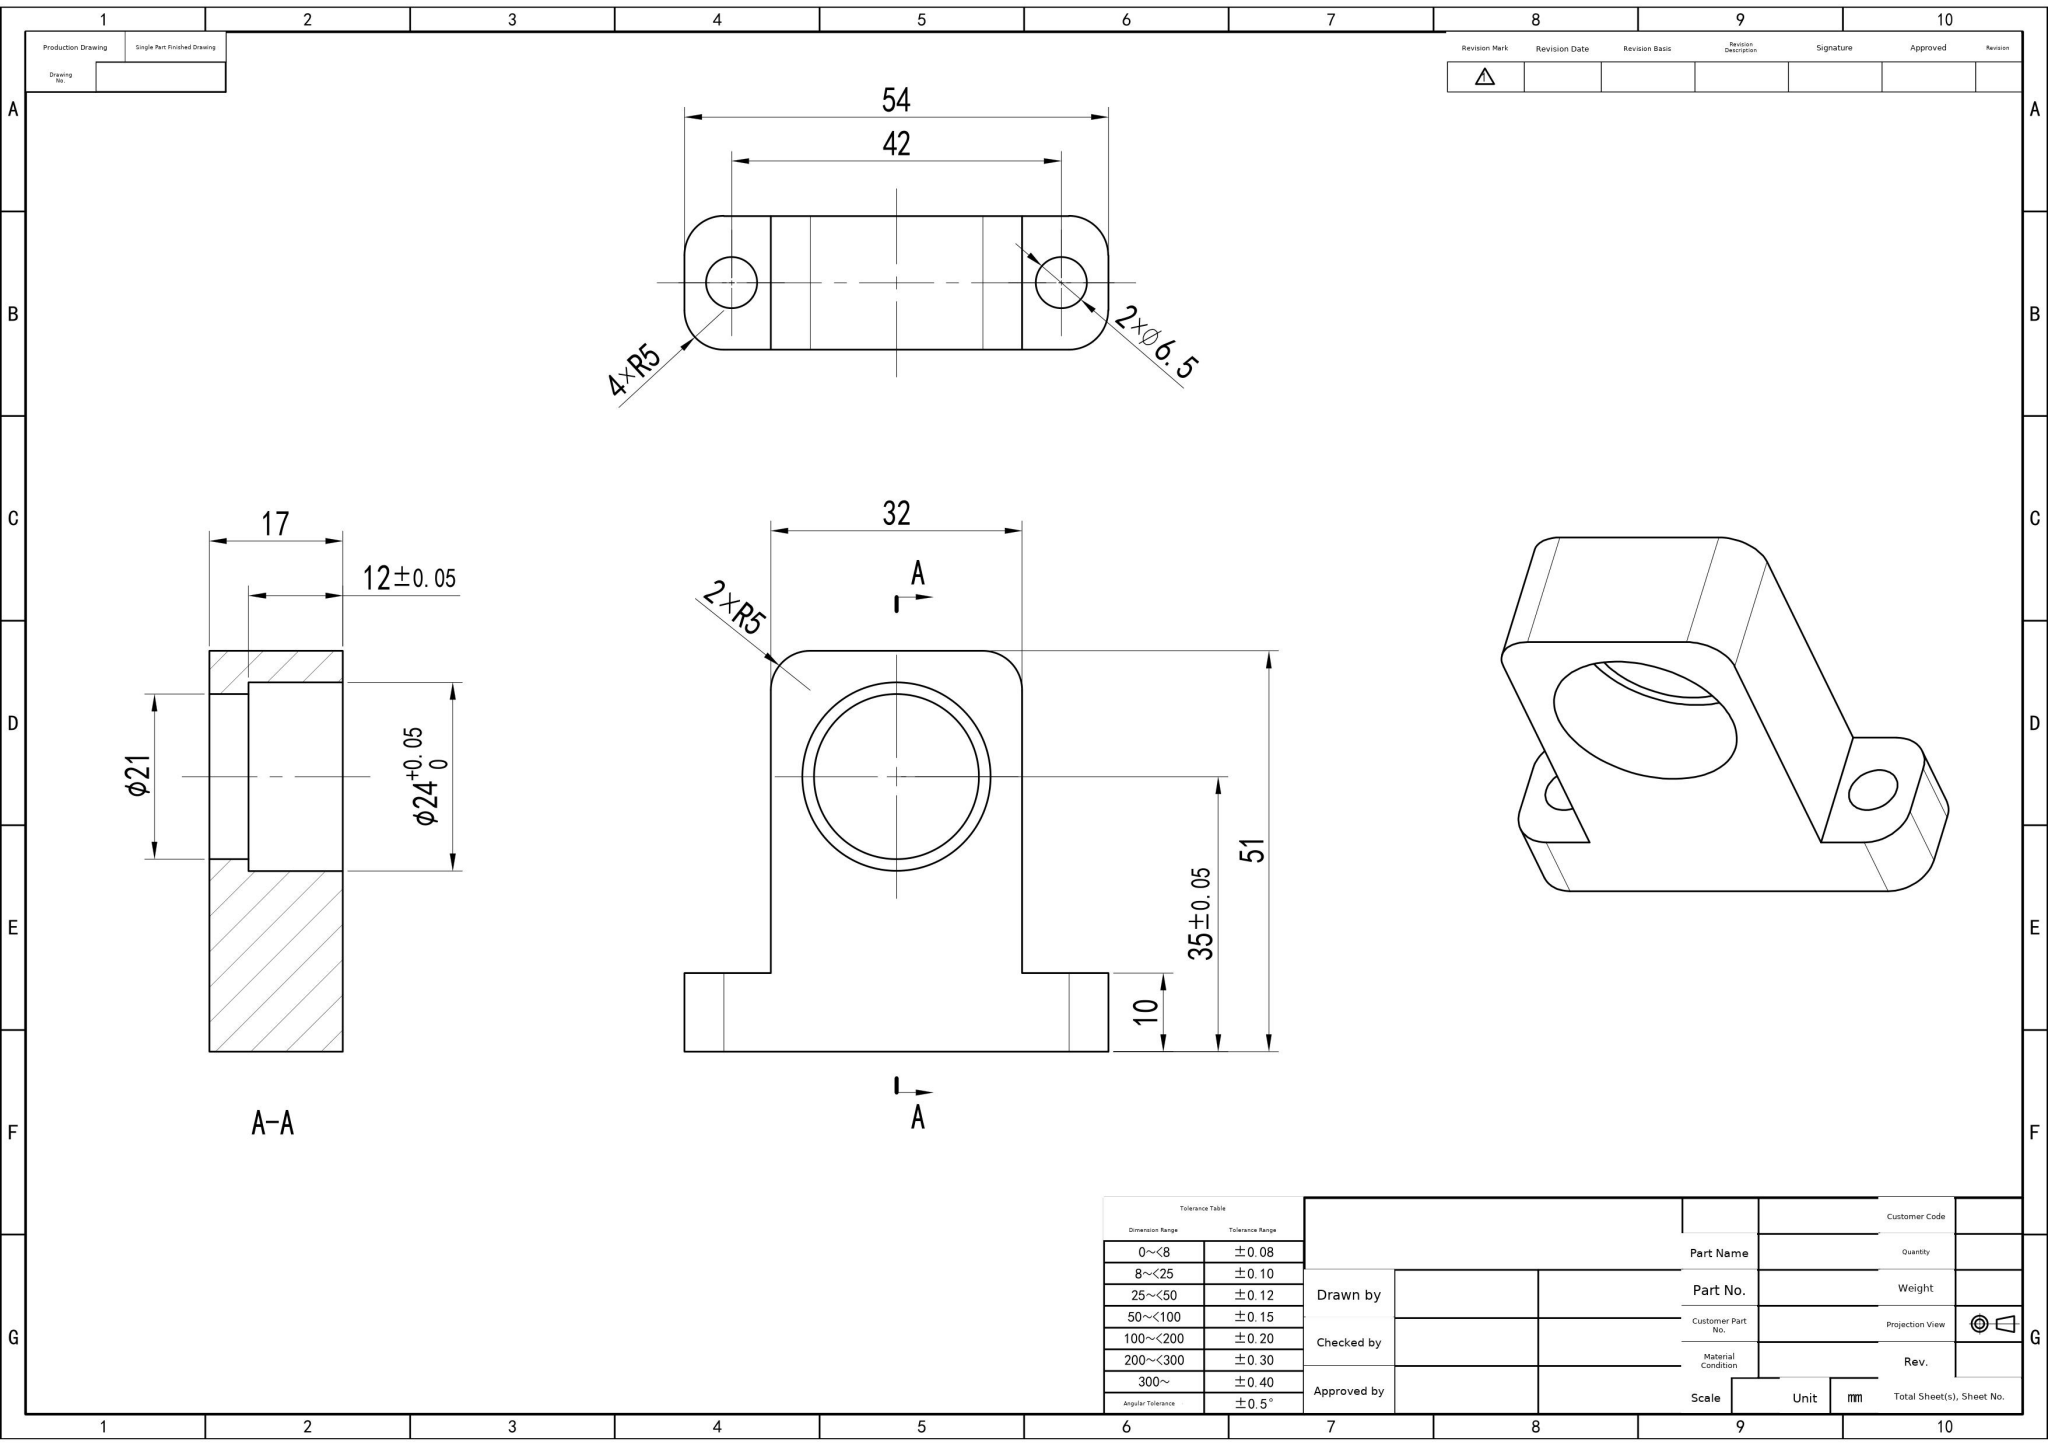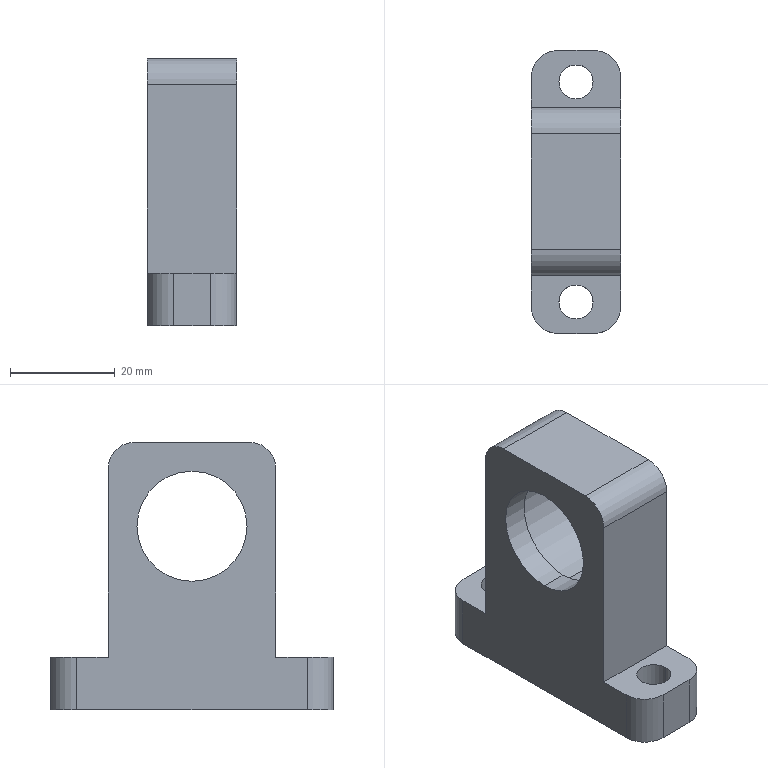Part | SolidWorks | mm | 1 solid | 25 faces | box 17 x 54 x 51 mm | volume 23263 mm3 | cylinder 14 | plane 11 | commonest cylinder face diameters 10 x6 6.5 x4 21 x2 24 x2
STEP:
#1=CARTESIAN_POINT('',(-3.5,0.,24.5));
#2=VERTEX_POINT('',#1);
#3=CARTESIAN_POINT('',(-3.5,0.,45.5));
#4=VERTEX_POINT('',#3);
#5=CARTESIAN_POINT('',(-3.5,0.,35.));
#6=DIRECTION('',(-1.,0.,0.));
#7=DIRECTION('',(0.,0.,1.));
#8=AXIS2_PLACEMENT_3D('',#5,#6,#7);
#9=CIRCLE('',#8,10.5);
#10=EDGE_CURVE('',#2,#4,#9,.T.);
#11=ORIENTED_EDGE('',*,*,#10,.F.);
#12=CARTESIAN_POINT('',(-8.5,0.,24.5));
#13=VERTEX_POINT('',#12);
#14=CARTESIAN_POINT('',(8.5,0.,24.5));
#15=DIRECTION('',(-1.,0.,0.));
#16=VECTOR('',#15,1000.);
#17=LINE('',#14,#16);
#18=EDGE_CURVE('',#2,#13,#17,.T.);
#19=ORIENTED_EDGE('',*,*,#18,.T.);
#20=CARTESIAN_POINT('',(-8.5,0.,45.5));
#21=VERTEX_POINT('',#20);
#22=CARTESIAN_POINT('',(-8.5,0.,35.));
#23=DIRECTION('',(-1.,0.,0.));
#24=DIRECTION('',(0.,0.,1.));
#25=AXIS2_PLACEMENT_3D('',#22,#23,#24);
#26=CIRCLE('',#25,10.5);
#27=EDGE_CURVE('',#13,#21,#26,.T.);
#28=ORIENTED_EDGE('',*,*,#27,.T.);
#29=CARTESIAN_POINT('',(8.5,0.,45.5));
#30=DIRECTION('',(-1.,0.,0.));
#31=VECTOR('',#30,1000.);
#32=LINE('',#29,#31);
#33=EDGE_CURVE('',#4,#21,#32,.T.);
#34=ORIENTED_EDGE('',*,*,#33,.F.);
#35=EDGE_LOOP('',(#11,#19,#28,#34));
#36=FACE_OUTER_BOUND('',#35,.T.);
#37=CARTESIAN_POINT('',(8.5,0.,35.));
#38=DIRECTION('',(-1.,0.,0.));
#39=DIRECTION('',(0.,0.,1.));
#40=AXIS2_PLACEMENT_3D('',#37,#38,#39);
#41=CYLINDRICAL_SURFACE('',#40,10.5);
#42=ADVANCED_FACE('',(#36),#41,.F.);
#43=CARTESIAN_POINT('',(3.25,21.,0.));
#44=VERTEX_POINT('',#43);
#45=CARTESIAN_POINT('',(-3.25,21.,0.));
#46=VERTEX_POINT('',#45);
#47=CARTESIAN_POINT('',(0.,21.,0.));
#48=DIRECTION('',(0.,0.,-1.));
#49=DIRECTION('',(1.,0.,0.));
#50=AXIS2_PLACEMENT_3D('',#47,#48,#49);
#51=CIRCLE('',#50,3.25);
#52=EDGE_CURVE('',#44,#46,#51,.T.);
#53=ORIENTED_EDGE('',*,*,#52,.T.);
#54=CARTESIAN_POINT('',(-3.25,21.,10.));
#55=VERTEX_POINT('',#54);
#56=CARTESIAN_POINT('',(-3.25,21.,0.));
#57=DIRECTION('',(0.,0.,1.));
#58=VECTOR('',#57,1000.);
#59=LINE('',#56,#58);
#60=EDGE_CURVE('',#46,#55,#59,.T.);
#61=ORIENTED_EDGE('',*,*,#60,.T.);
#62=CARTESIAN_POINT('',(3.25,21.,10.));
#63=VERTEX_POINT('',#62);
#64=CARTESIAN_POINT('',(0.,21.,10.));
#65=DIRECTION('',(0.,0.,1.));
#66=DIRECTION('',(1.,0.,0.));
#67=AXIS2_PLACEMENT_3D('',#64,#65,#66);
#68=CIRCLE('',#67,3.25);
#69=EDGE_CURVE('',#55,#63,#68,.T.);
#70=ORIENTED_EDGE('',*,*,#69,.T.);
#71=CARTESIAN_POINT('',(3.25,21.,0.));
#72=DIRECTION('',(0.,0.,1.));
#73=VECTOR('',#72,1000.);
#74=LINE('',#71,#73);
#75=EDGE_CURVE('',#44,#63,#74,.T.);
#76=ORIENTED_EDGE('',*,*,#75,.F.);
#77=EDGE_LOOP('',(#53,#61,#70,#76));
#78=FACE_OUTER_BOUND('',#77,.T.);
#79=CARTESIAN_POINT('',(0.,21.,0.));
#80=DIRECTION('',(0.,0.,1.));
#81=DIRECTION('',(1.,0.,0.));
#82=AXIS2_PLACEMENT_3D('',#79,#80,#81);
#83=CYLINDRICAL_SURFACE('',#82,3.25);
#84=ADVANCED_FACE('',(#78),#83,.F.);
#85=CARTESIAN_POINT('',(3.25,-21.,0.));
#86=VERTEX_POINT('',#85);
#87=CARTESIAN_POINT('',(-3.25,-21.,0.));
#88=VERTEX_POINT('',#87);
#89=CARTESIAN_POINT('',(-0.,-21.,0.));
#90=DIRECTION('',(0.,0.,-1.));
#91=DIRECTION('',(1.,0.,0.));
#92=AXIS2_PLACEMENT_3D('',#89,#90,#91);
#93=CIRCLE('',#92,3.25);
#94=EDGE_CURVE('',#86,#88,#93,.T.);
#95=ORIENTED_EDGE('',*,*,#94,.T.);
#96=CARTESIAN_POINT('',(-3.25,-21.,10.));
#97=VERTEX_POINT('',#96);
#98=CARTESIAN_POINT('',(-3.25,-21.,0.));
#99=DIRECTION('',(0.,0.,1.));
#100=VECTOR('',#99,1000.);
#101=LINE('',#98,#100);
#102=EDGE_CURVE('',#88,#97,#101,.T.);
#103=ORIENTED_EDGE('',*,*,#102,.T.);
#104=CARTESIAN_POINT('',(3.25,-21.,10.));
#105=VERTEX_POINT('',#104);
#106=CARTESIAN_POINT('',(-0.,-21.,10.));
#107=DIRECTION('',(0.,0.,1.));
#108=DIRECTION('',(1.,0.,0.));
#109=AXIS2_PLACEMENT_3D('',#106,#107,#108);
#110=CIRCLE('',#109,3.25);
#111=EDGE_CURVE('',#97,#105,#110,.T.);
#112=ORIENTED_EDGE('',*,*,#111,.T.);
#113=CARTESIAN_POINT('',(3.25,-21.,0.));
#114=DIRECTION('',(0.,0.,1.));
#115=VECTOR('',#114,1000.);
#116=LINE('',#113,#115);
#117=EDGE_CURVE('',#86,#105,#116,.T.);
#118=ORIENTED_EDGE('',*,*,#117,.F.);
#119=EDGE_LOOP('',(#95,#103,#112,#118));
#120=FACE_OUTER_BOUND('',#119,.T.);
#121=CARTESIAN_POINT('',(-0.,-21.,0.));
#122=DIRECTION('',(0.,0.,1.));
#123=DIRECTION('',(1.,0.,0.));
#124=AXIS2_PLACEMENT_3D('',#121,#122,#123);
#125=CYLINDRICAL_SURFACE('',#124,3.25);
#126=ADVANCED_FACE('',(#120),#125,.F.);
#127=CARTESIAN_POINT('',(8.5,0.,23.));
#128=VERTEX_POINT('',#127);
#129=CARTESIAN_POINT('',(8.5,0.,47.));
#130=VERTEX_POINT('',#129);
#131=CARTESIAN_POINT('',(8.5,0.,35.));
#132=DIRECTION('',(-1.,0.,0.));
#133=DIRECTION('',(0.,0.,1.));
#134=AXIS2_PLACEMENT_3D('',#131,#132,#133);
#135=CIRCLE('',#134,12.);
#136=EDGE_CURVE('',#128,#130,#135,.T.);
#137=ORIENTED_EDGE('',*,*,#136,.F.);
#138=CARTESIAN_POINT('',(-3.5,0.,23.));
#139=VERTEX_POINT('',#138);
#140=CARTESIAN_POINT('',(8.5,0.,23.));
#141=DIRECTION('',(-1.,0.,0.));
#142=VECTOR('',#141,1000.);
#143=LINE('',#140,#142);
#144=EDGE_CURVE('',#128,#139,#143,.T.);
#145=ORIENTED_EDGE('',*,*,#144,.T.);
#146=CARTESIAN_POINT('',(-3.5,0.,47.));
#147=VERTEX_POINT('',#146);
#148=CARTESIAN_POINT('',(-3.5,0.,35.));
#149=DIRECTION('',(-1.,0.,0.));
#150=DIRECTION('',(0.,0.,1.));
#151=AXIS2_PLACEMENT_3D('',#148,#149,#150);
#152=CIRCLE('',#151,12.);
#153=EDGE_CURVE('',#139,#147,#152,.T.);
#154=ORIENTED_EDGE('',*,*,#153,.T.);
#155=CARTESIAN_POINT('',(8.5,0.,47.));
#156=DIRECTION('',(-1.,0.,0.));
#157=VECTOR('',#156,1000.);
#158=LINE('',#155,#157);
#159=EDGE_CURVE('',#130,#147,#158,.T.);
#160=ORIENTED_EDGE('',*,*,#159,.F.);
#161=EDGE_LOOP('',(#137,#145,#154,#160));
#162=FACE_OUTER_BOUND('',#161,.T.);
#163=CARTESIAN_POINT('',(8.5,0.,35.));
#164=DIRECTION('',(-1.,0.,0.));
#165=DIRECTION('',(0.,0.,1.));
#166=AXIS2_PLACEMENT_3D('',#163,#164,#165);
#167=CYLINDRICAL_SURFACE('',#166,12.);
#168=ADVANCED_FACE('',(#162),#167,.F.);
#169=CARTESIAN_POINT('',(-8.5,0.,35.));
#170=DIRECTION('',(-1.,0.,0.));
#171=DIRECTION('',(0.,0.,1.));
#172=AXIS2_PLACEMENT_3D('',#169,#170,#171);
#173=CIRCLE('',#172,10.5);
#174=EDGE_CURVE('',#21,#13,#173,.T.);
#175=ORIENTED_EDGE('',*,*,#174,.F.);
#176=ORIENTED_EDGE('',*,*,#27,.F.);
#177=EDGE_LOOP('',(#175,#176));
#178=FACE_BOUND('',#177,.T.);
#179=CARTESIAN_POINT('',(-8.5,22.,-0.));
#180=VERTEX_POINT('',#179);
#181=CARTESIAN_POINT('',(-8.5,22.,10.));
#182=VERTEX_POINT('',#181);
#183=CARTESIAN_POINT('',(-8.5,22.,46.));
#184=DIRECTION('',(0.,0.,1.));
#185=VECTOR('',#184,1000.);
#186=LINE('',#183,#185);
#187=EDGE_CURVE('',#180,#182,#186,.T.);
#188=ORIENTED_EDGE('',*,*,#187,.F.);
#189=CARTESIAN_POINT('',(-8.5,-22.,0.));
#190=VERTEX_POINT('',#189);
#191=CARTESIAN_POINT('',(-8.5,11.,0.));
#192=DIRECTION('',(0.,1.,0.));
#193=VECTOR('',#192,1000.);
#194=LINE('',#191,#193);
#195=EDGE_CURVE('',#190,#180,#194,.T.);
#196=ORIENTED_EDGE('',*,*,#195,.F.);
#197=CARTESIAN_POINT('',(-8.5,-22.,10.));
#198=VERTEX_POINT('',#197);
#199=CARTESIAN_POINT('',(-8.5,-22.,46.));
#200=DIRECTION('',(0.,0.,-1.));
#201=VECTOR('',#200,1000.);
#202=LINE('',#199,#201);
#203=EDGE_CURVE('',#198,#190,#202,.T.);
#204=ORIENTED_EDGE('',*,*,#203,.F.);
#205=CARTESIAN_POINT('',(-8.5,-16.,10.));
#206=VERTEX_POINT('',#205);
#207=CARTESIAN_POINT('',(-8.5,11.,10.));
#208=DIRECTION('',(0.,-1.,0.));
#209=VECTOR('',#208,1000.);
#210=LINE('',#207,#209);
#211=EDGE_CURVE('',#206,#198,#210,.T.);
#212=ORIENTED_EDGE('',*,*,#211,.F.);
#213=CARTESIAN_POINT('',(-8.5,-16.,46.));
#214=VERTEX_POINT('',#213);
#215=CARTESIAN_POINT('',(-8.5,-16.,46.));
#216=DIRECTION('',(0.,0.,-1.));
#217=VECTOR('',#216,1000.);
#218=LINE('',#215,#217);
#219=EDGE_CURVE('',#214,#206,#218,.T.);
#220=ORIENTED_EDGE('',*,*,#219,.F.);
#221=CARTESIAN_POINT('',(-8.5,-11.,51.));
#222=VERTEX_POINT('',#221);
#223=CARTESIAN_POINT('',(-8.5,-11.,46.));
#224=DIRECTION('',(1.,0.,0.));
#225=DIRECTION('',(0.,0.,1.));
#226=AXIS2_PLACEMENT_3D('',#223,#224,#225);
#227=CIRCLE('',#226,5.);
#228=EDGE_CURVE('',#222,#214,#227,.T.);
#229=ORIENTED_EDGE('',*,*,#228,.F.);
#230=CARTESIAN_POINT('',(-8.5,11.,51.));
#231=VERTEX_POINT('',#230);
#232=CARTESIAN_POINT('',(-8.5,11.,51.));
#233=DIRECTION('',(0.,-1.,0.));
#234=VECTOR('',#233,1000.);
#235=LINE('',#232,#234);
#236=EDGE_CURVE('',#231,#222,#235,.T.);
#237=ORIENTED_EDGE('',*,*,#236,.F.);
#238=CARTESIAN_POINT('',(-8.5,16.,46.));
#239=VERTEX_POINT('',#238);
#240=CARTESIAN_POINT('',(-8.5,11.,46.));
#241=DIRECTION('',(1.,0.,0.));
#242=DIRECTION('',(0.,0.,1.));
#243=AXIS2_PLACEMENT_3D('',#240,#241,#242);
#244=CIRCLE('',#243,5.);
#245=EDGE_CURVE('',#239,#231,#244,.T.);
#246=ORIENTED_EDGE('',*,*,#245,.F.);
#247=CARTESIAN_POINT('',(-8.5,16.,10.));
#248=VERTEX_POINT('',#247);
#249=CARTESIAN_POINT('',(-8.5,16.,46.));
#250=DIRECTION('',(0.,0.,1.));
#251=VECTOR('',#250,1000.);
#252=LINE('',#249,#251);
#253=EDGE_CURVE('',#248,#239,#252,.T.);
#254=ORIENTED_EDGE('',*,*,#253,.F.);
#255=CARTESIAN_POINT('',(-8.5,11.,10.));
#256=DIRECTION('',(0.,-1.,0.));
#257=VECTOR('',#256,1000.);
#258=LINE('',#255,#257);
#259=EDGE_CURVE('',#182,#248,#258,.T.);
#260=ORIENTED_EDGE('',*,*,#259,.F.);
#261=EDGE_LOOP('',(#188,#196,#204,#212,#220,#229,#237,#246,#254,#260));
#262=FACE_OUTER_BOUND('',#261,.T.);
#263=CARTESIAN_POINT('',(-8.5,11.,46.));
#264=DIRECTION('',(1.,0.,0.));
#265=DIRECTION('',(0.,0.,-1.));
#266=AXIS2_PLACEMENT_3D('',#263,#264,#265);
#267=PLANE('',#266);
#268=ADVANCED_FACE('',(#178,#262),#267,.F.);
#269=ORIENTED_EDGE('',*,*,#18,.F.);
#270=CARTESIAN_POINT('',(-3.5,0.,35.));
#271=DIRECTION('',(-1.,0.,0.));
#272=DIRECTION('',(0.,0.,1.));
#273=AXIS2_PLACEMENT_3D('',#270,#271,#272);
#274=CIRCLE('',#273,10.5);
#275=EDGE_CURVE('',#4,#2,#274,.T.);
#276=ORIENTED_EDGE('',*,*,#275,.F.);
#277=ORIENTED_EDGE('',*,*,#33,.T.);
#278=ORIENTED_EDGE('',*,*,#174,.T.);
#279=EDGE_LOOP('',(#269,#276,#277,#278));
#280=FACE_OUTER_BOUND('',#279,.T.);
#281=CARTESIAN_POINT('',(8.5,0.,35.));
#282=DIRECTION('',(-1.,0.,0.));
#283=DIRECTION('',(0.,0.,1.));
#284=AXIS2_PLACEMENT_3D('',#281,#282,#283);
#285=CYLINDRICAL_SURFACE('',#284,10.5);
#286=ADVANCED_FACE('',(#280),#285,.F.);
#287=CARTESIAN_POINT('',(3.5,27.,10.));
#288=VERTEX_POINT('',#287);
#289=CARTESIAN_POINT('',(8.5,22.,10.));
#290=VERTEX_POINT('',#289);
#291=CARTESIAN_POINT('',(3.5,22.,10.));
#292=DIRECTION('',(0.,0.,-1.));
#293=DIRECTION('',(0.,1.,0.));
#294=AXIS2_PLACEMENT_3D('',#291,#292,#293);
#295=CIRCLE('',#294,5.);
#296=EDGE_CURVE('',#288,#290,#295,.T.);
#297=ORIENTED_EDGE('',*,*,#296,.F.);
#298=CARTESIAN_POINT('',(-3.5,27.,10.));
#299=VERTEX_POINT('',#298);
#300=CARTESIAN_POINT('',(8.5,27.,10.));
#301=DIRECTION('',(1.,0.,0.));
#302=VECTOR('',#301,1000.);
#303=LINE('',#300,#302);
#304=EDGE_CURVE('',#299,#288,#303,.T.);
#305=ORIENTED_EDGE('',*,*,#304,.F.);
#306=CARTESIAN_POINT('',(-3.5,22.,10.));
#307=DIRECTION('',(0.,0.,-1.));
#308=DIRECTION('',(0.,-1.,-0.));
#309=AXIS2_PLACEMENT_3D('',#306,#307,#308);
#310=CIRCLE('',#309,5.);
#311=EDGE_CURVE('',#182,#299,#310,.T.);
#312=ORIENTED_EDGE('',*,*,#311,.F.);
#313=ORIENTED_EDGE('',*,*,#259,.T.);
#314=CARTESIAN_POINT('',(8.5,16.,10.));
#315=VERTEX_POINT('',#314);
#316=CARTESIAN_POINT('',(8.5,16.,10.));
#317=DIRECTION('',(-1.,0.,0.));
#318=VECTOR('',#317,1000.);
#319=LINE('',#316,#318);
#320=EDGE_CURVE('',#315,#248,#319,.T.);
#321=ORIENTED_EDGE('',*,*,#320,.F.);
#322=CARTESIAN_POINT('',(8.5,27.,10.));
#323=DIRECTION('',(0.,-1.,0.));
#324=VECTOR('',#323,1000.);
#325=LINE('',#322,#324);
#326=EDGE_CURVE('',#290,#315,#325,.T.);
#327=ORIENTED_EDGE('',*,*,#326,.F.);
#328=EDGE_LOOP('',(#297,#305,#312,#313,#321,#327));
#329=FACE_OUTER_BOUND('',#328,.T.);
#330=CARTESIAN_POINT('',(0.,21.,10.));
#331=DIRECTION('',(0.,0.,1.));
#332=DIRECTION('',(1.,0.,0.));
#333=AXIS2_PLACEMENT_3D('',#330,#331,#332);
#334=CIRCLE('',#333,3.25);
#335=EDGE_CURVE('',#63,#55,#334,.T.);
#336=ORIENTED_EDGE('',*,*,#335,.F.);
#337=ORIENTED_EDGE('',*,*,#69,.F.);
#338=EDGE_LOOP('',(#336,#337));
#339=FACE_BOUND('',#338,.T.);
#340=CARTESIAN_POINT('',(8.5,27.,10.));
#341=DIRECTION('',(0.,0.,-1.));
#342=DIRECTION('',(-1.,0.,0.));
#343=AXIS2_PLACEMENT_3D('',#340,#341,#342);
#344=PLANE('',#343);
#345=ADVANCED_FACE('',(#329,#339),#344,.F.);
#346=ORIENTED_EDGE('',*,*,#311,.T.);
#347=CARTESIAN_POINT('',(-3.5,27.,-0.));
#348=VERTEX_POINT('',#347);
#349=CARTESIAN_POINT('',(-3.5,27.,0.));
#350=DIRECTION('',(0.,0.,-1.));
#351=VECTOR('',#350,1000.);
#352=LINE('',#349,#351);
#353=EDGE_CURVE('',#299,#348,#352,.T.);
#354=ORIENTED_EDGE('',*,*,#353,.T.);
#355=CARTESIAN_POINT('',(-3.5,22.,-0.));
#356=DIRECTION('',(0.,-0.,1.));
#357=DIRECTION('',(0.,-1.,-0.));
#358=AXIS2_PLACEMENT_3D('',#355,#356,#357);
#359=CIRCLE('',#358,5.);
#360=EDGE_CURVE('',#348,#180,#359,.T.);
#361=ORIENTED_EDGE('',*,*,#360,.T.);
#362=ORIENTED_EDGE('',*,*,#187,.T.);
#363=EDGE_LOOP('',(#346,#354,#361,#362));
#364=FACE_OUTER_BOUND('',#363,.T.);
#365=CARTESIAN_POINT('',(-3.5,22.,-0.));
#366=DIRECTION('',(0.,-0.,1.));
#367=DIRECTION('',(0.,-1.,-0.));
#368=AXIS2_PLACEMENT_3D('',#365,#366,#367);
#369=CYLINDRICAL_SURFACE('',#368,5.);
#370=ADVANCED_FACE('',(#364),#369,.T.);
#371=CARTESIAN_POINT('',(8.5,22.,0.));
#372=VERTEX_POINT('',#371);
#373=CARTESIAN_POINT('',(3.5,27.,0.));
#374=VERTEX_POINT('',#373);
#375=CARTESIAN_POINT('',(3.5,22.,0.));
#376=DIRECTION('',(0.,-0.,1.));
#377=DIRECTION('',(0.,1.,0.));
#378=AXIS2_PLACEMENT_3D('',#375,#376,#377);
#379=CIRCLE('',#378,5.);
#380=EDGE_CURVE('',#372,#374,#379,.T.);
#381=ORIENTED_EDGE('',*,*,#380,.F.);
#382=CARTESIAN_POINT('',(8.5,-22.,-0.));
#383=VERTEX_POINT('',#382);
#384=CARTESIAN_POINT('',(8.5,-27.,0.));
#385=DIRECTION('',(0.,1.,0.));
#386=VECTOR('',#385,1000.);
#387=LINE('',#384,#386);
#388=EDGE_CURVE('',#383,#372,#387,.T.);
#389=ORIENTED_EDGE('',*,*,#388,.F.);
#390=CARTESIAN_POINT('',(3.5,-27.,-0.));
#391=VERTEX_POINT('',#390);
#392=CARTESIAN_POINT('',(3.5,-22.,-0.));
#393=DIRECTION('',(0.,0.,1.));
#394=DIRECTION('',(0.,-1.,0.));
#395=AXIS2_PLACEMENT_3D('',#392,#393,#394);
#396=CIRCLE('',#395,5.);
#397=EDGE_CURVE('',#391,#383,#396,.T.);
#398=ORIENTED_EDGE('',*,*,#397,.F.);
#399=CARTESIAN_POINT('',(-3.5,-27.,0.));
#400=VERTEX_POINT('',#399);
#401=CARTESIAN_POINT('',(8.5,-27.,0.));
#402=DIRECTION('',(1.,0.,0.));
#403=VECTOR('',#402,1000.);
#404=LINE('',#401,#403);
#405=EDGE_CURVE('',#400,#391,#404,.T.);
#406=ORIENTED_EDGE('',*,*,#405,.F.);
#407=CARTESIAN_POINT('',(-3.5,-22.,0.));
#408=DIRECTION('',(0.,0.,1.));
#409=DIRECTION('',(0.,1.,-0.));
#410=AXIS2_PLACEMENT_3D('',#407,#408,#409);
#411=CIRCLE('',#410,5.);
#412=EDGE_CURVE('',#190,#400,#411,.T.);
#413=ORIENTED_EDGE('',*,*,#412,.F.);
#414=ORIENTED_EDGE('',*,*,#195,.T.);
#415=ORIENTED_EDGE('',*,*,#360,.F.);
#416=CARTESIAN_POINT('',(8.5,27.,0.));
#417=DIRECTION('',(-1.,0.,0.));
#418=VECTOR('',#417,1000.);
#419=LINE('',#416,#418);
#420=EDGE_CURVE('',#374,#348,#419,.T.);
#421=ORIENTED_EDGE('',*,*,#420,.F.);
#422=EDGE_LOOP('',(#381,#389,#398,#406,#413,#414,#415,#421));
#423=FACE_OUTER_BOUND('',#422,.T.);
#424=ORIENTED_EDGE('',*,*,#94,.F.);
#425=CARTESIAN_POINT('',(-0.,-21.,0.));
#426=DIRECTION('',(0.,0.,-1.));
#427=DIRECTION('',(1.,0.,0.));
#428=AXIS2_PLACEMENT_3D('',#425,#426,#427);
#429=CIRCLE('',#428,3.25);
#430=EDGE_CURVE('',#88,#86,#429,.T.);
#431=ORIENTED_EDGE('',*,*,#430,.F.);
#432=EDGE_LOOP('',(#424,#431));
#433=FACE_BOUND('',#432,.T.);
#434=ORIENTED_EDGE('',*,*,#52,.F.);
#435=CARTESIAN_POINT('',(0.,21.,0.));
#436=DIRECTION('',(0.,0.,-1.));
#437=DIRECTION('',(1.,0.,0.));
#438=AXIS2_PLACEMENT_3D('',#435,#436,#437);
#439=CIRCLE('',#438,3.25);
#440=EDGE_CURVE('',#46,#44,#439,.T.);
#441=ORIENTED_EDGE('',*,*,#440,.F.);
#442=EDGE_LOOP('',(#434,#441));
#443=FACE_BOUND('',#442,.T.);
#444=CARTESIAN_POINT('',(8.5,-27.,0.));
#445=DIRECTION('',(0.,0.,1.));
#446=DIRECTION('',(1.,0.,0.));
#447=AXIS2_PLACEMENT_3D('',#444,#445,#446);
#448=PLANE('',#447);
#449=ADVANCED_FACE('',(#423,#433,#443),#448,.F.);
#450=ORIENTED_EDGE('',*,*,#412,.T.);
#451=CARTESIAN_POINT('',(-3.5,-27.,10.));
#452=VERTEX_POINT('',#451);
#453=CARTESIAN_POINT('',(-3.5,-27.,10.));
#454=DIRECTION('',(0.,0.,1.));
#455=VECTOR('',#454,1000.);
#456=LINE('',#453,#455);
#457=EDGE_CURVE('',#400,#452,#456,.T.);
#458=ORIENTED_EDGE('',*,*,#457,.T.);
#459=CARTESIAN_POINT('',(-3.5,-22.,10.));
#460=DIRECTION('',(0.,-0.,-1.));
#461=DIRECTION('',(0.,1.,-0.));
#462=AXIS2_PLACEMENT_3D('',#459,#460,#461);
#463=CIRCLE('',#462,5.);
#464=EDGE_CURVE('',#452,#198,#463,.T.);
#465=ORIENTED_EDGE('',*,*,#464,.T.);
#466=ORIENTED_EDGE('',*,*,#203,.T.);
#467=EDGE_LOOP('',(#450,#458,#465,#466));
#468=FACE_OUTER_BOUND('',#467,.T.);
#469=CARTESIAN_POINT('',(-3.5,-22.,10.));
#470=DIRECTION('',(0.,-0.,-1.));
#471=DIRECTION('',(0.,1.,-0.));
#472=AXIS2_PLACEMENT_3D('',#469,#470,#471);
#473=CYLINDRICAL_SURFACE('',#472,5.);
#474=ADVANCED_FACE('',(#468),#473,.T.);
#475=CARTESIAN_POINT('',(8.5,-22.,10.));
#476=VERTEX_POINT('',#475);
#477=CARTESIAN_POINT('',(3.5,-27.,10.));
#478=VERTEX_POINT('',#477);
#479=CARTESIAN_POINT('',(3.5,-22.,10.));
#480=DIRECTION('',(0.,-0.,-1.));
#481=DIRECTION('',(-0.,-1.,0.));
#482=AXIS2_PLACEMENT_3D('',#479,#480,#481);
#483=CIRCLE('',#482,5.);
#484=EDGE_CURVE('',#476,#478,#483,.T.);
#485=ORIENTED_EDGE('',*,*,#484,.F.);
#486=CARTESIAN_POINT('',(8.5,-16.,10.));
#487=VERTEX_POINT('',#486);
#488=CARTESIAN_POINT('',(8.5,-16.,10.));
#489=DIRECTION('',(0.,-1.,0.));
#490=VECTOR('',#489,1000.);
#491=LINE('',#488,#490);
#492=EDGE_CURVE('',#487,#476,#491,.T.);
#493=ORIENTED_EDGE('',*,*,#492,.F.);
#494=CARTESIAN_POINT('',(8.5,-16.,10.));
#495=DIRECTION('',(1.,0.,0.));
#496=VECTOR('',#495,1000.);
#497=LINE('',#494,#496);
#498=EDGE_CURVE('',#206,#487,#497,.T.);
#499=ORIENTED_EDGE('',*,*,#498,.F.);
#500=ORIENTED_EDGE('',*,*,#211,.T.);
#501=ORIENTED_EDGE('',*,*,#464,.F.);
#502=CARTESIAN_POINT('',(8.5,-27.,10.));
#503=DIRECTION('',(-1.,0.,0.));
#504=VECTOR('',#503,1000.);
#505=LINE('',#502,#504);
#506=EDGE_CURVE('',#478,#452,#505,.T.);
#507=ORIENTED_EDGE('',*,*,#506,.F.);
#508=EDGE_LOOP('',(#485,#493,#499,#500,#501,#507));
#509=FACE_OUTER_BOUND('',#508,.T.);
#510=CARTESIAN_POINT('',(-0.,-21.,10.));
#511=DIRECTION('',(0.,0.,1.));
#512=DIRECTION('',(1.,0.,0.));
#513=AXIS2_PLACEMENT_3D('',#510,#511,#512);
#514=CIRCLE('',#513,3.25);
#515=EDGE_CURVE('',#105,#97,#514,.T.);
#516=ORIENTED_EDGE('',*,*,#515,.F.);
#517=ORIENTED_EDGE('',*,*,#111,.F.);
#518=EDGE_LOOP('',(#516,#517));
#519=FACE_BOUND('',#518,.T.);
#520=CARTESIAN_POINT('',(8.5,-16.,10.));
#521=DIRECTION('',(0.,0.,-1.));
#522=DIRECTION('',(-1.,0.,0.));
#523=AXIS2_PLACEMENT_3D('',#520,#521,#522);
#524=PLANE('',#523);
#525=ADVANCED_FACE('',(#509,#519),#524,.F.);
#526=ORIENTED_EDGE('',*,*,#498,.T.);
#527=CARTESIAN_POINT('',(8.5,-16.,46.));
#528=VERTEX_POINT('',#527);
#529=CARTESIAN_POINT('',(8.5,-16.,46.));
#530=DIRECTION('',(0.,0.,-1.));
#531=VECTOR('',#530,1000.);
#532=LINE('',#529,#531);
#533=EDGE_CURVE('',#528,#487,#532,.T.);
#534=ORIENTED_EDGE('',*,*,#533,.F.);
#535=CARTESIAN_POINT('',(8.5,-16.,46.));
#536=DIRECTION('',(1.,0.,0.));
#537=VECTOR('',#536,1000.);
#538=LINE('',#535,#537);
#539=EDGE_CURVE('',#214,#528,#538,.T.);
#540=ORIENTED_EDGE('',*,*,#539,.F.);
#541=ORIENTED_EDGE('',*,*,#219,.T.);
#542=EDGE_LOOP('',(#526,#534,#540,#541));
#543=FACE_OUTER_BOUND('',#542,.T.);
#544=CARTESIAN_POINT('',(8.5,-16.,46.));
#545=DIRECTION('',(0.,1.,0.));
#546=DIRECTION('',(0.,0.,1.));
#547=AXIS2_PLACEMENT_3D('',#544,#545,#546);
#548=PLANE('',#547);
#549=ADVANCED_FACE('',(#543),#548,.F.);
#550=CARTESIAN_POINT('',(8.5,-11.,51.));
#551=VERTEX_POINT('',#550);
#552=CARTESIAN_POINT('',(8.5,-11.,46.));
#553=DIRECTION('',(-1.,0.,0.));
#554=DIRECTION('',(0.,0.,1.));
#555=AXIS2_PLACEMENT_3D('',#552,#553,#554);
#556=CIRCLE('',#555,5.);
#557=EDGE_CURVE('',#528,#551,#556,.T.);
#558=ORIENTED_EDGE('',*,*,#557,.T.);
#559=CARTESIAN_POINT('',(8.5,-11.,51.));
#560=DIRECTION('',(-1.,0.,0.));
#561=VECTOR('',#560,1000.);
#562=LINE('',#559,#561);
#563=EDGE_CURVE('',#551,#222,#562,.T.);
#564=ORIENTED_EDGE('',*,*,#563,.T.);
#565=ORIENTED_EDGE('',*,*,#228,.T.);
#566=ORIENTED_EDGE('',*,*,#539,.T.);
#567=EDGE_LOOP('',(#558,#564,#565,#566));
#568=FACE_OUTER_BOUND('',#567,.T.);
#569=CARTESIAN_POINT('',(8.5,-11.,46.));
#570=DIRECTION('',(-1.,0.,0.));
#571=DIRECTION('',(0.,0.,1.));
#572=AXIS2_PLACEMENT_3D('',#569,#570,#571);
#573=CYLINDRICAL_SURFACE('',#572,5.);
#574=ADVANCED_FACE('',(#568),#573,.T.);
#575=ORIENTED_EDGE('',*,*,#563,.F.);
#576=CARTESIAN_POINT('',(8.5,11.,51.));
#577=VERTEX_POINT('',#576);
#578=CARTESIAN_POINT('',(8.5,11.,51.));
#579=DIRECTION('',(0.,-1.,0.));
#580=VECTOR('',#579,1000.);
#581=LINE('',#578,#580);
#582=EDGE_CURVE('',#577,#551,#581,.T.);
#583=ORIENTED_EDGE('',*,*,#582,.F.);
#584=CARTESIAN_POINT('',(8.5,11.,51.));
#585=DIRECTION('',(1.,0.,0.));
#586=VECTOR('',#585,1000.);
#587=LINE('',#584,#586);
#588=EDGE_CURVE('',#231,#577,#587,.T.);
#589=ORIENTED_EDGE('',*,*,#588,.F.);
#590=ORIENTED_EDGE('',*,*,#236,.T.);
#591=EDGE_LOOP('',(#575,#583,#589,#590));
#592=FACE_OUTER_BOUND('',#591,.T.);
#593=CARTESIAN_POINT('',(8.5,11.,51.));
#594=DIRECTION('',(0.,-0.,-1.));
#595=DIRECTION('',(0.,1.,-0.));
#596=AXIS2_PLACEMENT_3D('',#593,#594,#595);
#597=PLANE('',#596);
#598=ADVANCED_FACE('',(#592),#597,.F.);
#599=CARTESIAN_POINT('',(8.5,16.,46.));
#600=VERTEX_POINT('',#599);
#601=CARTESIAN_POINT('',(8.5,11.,46.));
#602=DIRECTION('',(-1.,0.,0.));
#603=DIRECTION('',(0.,0.,1.));
#604=AXIS2_PLACEMENT_3D('',#601,#602,#603);
#605=CIRCLE('',#604,5.);
#606=EDGE_CURVE('',#577,#600,#605,.T.);
#607=ORIENTED_EDGE('',*,*,#606,.T.);
#608=CARTESIAN_POINT('',(8.5,16.,46.));
#609=DIRECTION('',(-1.,0.,0.));
#610=VECTOR('',#609,1000.);
#611=LINE('',#608,#610);
#612=EDGE_CURVE('',#600,#239,#611,.T.);
#613=ORIENTED_EDGE('',*,*,#612,.T.);
#614=ORIENTED_EDGE('',*,*,#245,.T.);
#615=ORIENTED_EDGE('',*,*,#588,.T.);
#616=EDGE_LOOP('',(#607,#613,#614,#615));
#617=FACE_OUTER_BOUND('',#616,.T.);
#618=CARTESIAN_POINT('',(8.5,11.,46.));
#619=DIRECTION('',(-1.,0.,0.));
#620=DIRECTION('',(0.,0.,1.));
#621=AXIS2_PLACEMENT_3D('',#618,#619,#620);
#622=CYLINDRICAL_SURFACE('',#621,5.);
#623=ADVANCED_FACE('',(#617),#622,.T.);
#624=ORIENTED_EDGE('',*,*,#612,.F.);
#625=CARTESIAN_POINT('',(8.5,16.,10.));
#626=DIRECTION('',(0.,0.,1.));
#627=VECTOR('',#626,1000.);
#628=LINE('',#625,#627);
#629=EDGE_CURVE('',#315,#600,#628,.T.);
#630=ORIENTED_EDGE('',*,*,#629,.F.);
#631=ORIENTED_EDGE('',*,*,#320,.T.);
#632=ORIENTED_EDGE('',*,*,#253,.T.);
#633=EDGE_LOOP('',(#624,#630,#631,#632));
#634=FACE_OUTER_BOUND('',#633,.T.);
#635=CARTESIAN_POINT('',(8.5,16.,10.));
#636=DIRECTION('',(0.,-1.,0.));
#637=DIRECTION('',(0.,0.,-1.));
#638=AXIS2_PLACEMENT_3D('',#635,#636,#637);
#639=PLANE('',#638);
#640=ADVANCED_FACE('',(#634),#639,.F.);
#641=CARTESIAN_POINT('',(-3.5,0.,35.));
#642=DIRECTION('',(-1.,0.,0.));
#643=DIRECTION('',(0.,0.,1.));
#644=AXIS2_PLACEMENT_3D('',#641,#642,#643);
#645=CIRCLE('',#644,12.);
#646=EDGE_CURVE('',#147,#139,#645,.T.);
#647=ORIENTED_EDGE('',*,*,#646,.F.);
#648=ORIENTED_EDGE('',*,*,#153,.F.);
#649=EDGE_LOOP('',(#647,#648));
#650=FACE_OUTER_BOUND('',#649,.T.);
#651=ORIENTED_EDGE('',*,*,#275,.T.);
#652=ORIENTED_EDGE('',*,*,#10,.T.);
#653=EDGE_LOOP('',(#651,#652));
#654=FACE_BOUND('',#653,.T.);
#655=CARTESIAN_POINT('',(-3.5,0.,35.));
#656=DIRECTION('',(-1.,0.,0.));
#657=DIRECTION('',(0.,0.,1.));
#658=AXIS2_PLACEMENT_3D('',#655,#656,#657);
#659=PLANE('',#658);
#660=ADVANCED_FACE('',(#650,#654),#659,.F.);
#661=ORIENTED_EDGE('',*,*,#492,.T.);
#662=CARTESIAN_POINT('',(8.5,-22.,46.));
#663=DIRECTION('',(0.,0.,-1.));
#664=VECTOR('',#663,1000.);
#665=LINE('',#662,#664);
#666=EDGE_CURVE('',#476,#383,#665,.T.);
#667=ORIENTED_EDGE('',*,*,#666,.T.);
#668=ORIENTED_EDGE('',*,*,#388,.T.);
#669=CARTESIAN_POINT('',(8.5,22.,46.));
#670=DIRECTION('',(0.,0.,1.));
#671=VECTOR('',#670,1000.);
#672=LINE('',#669,#671);
#673=EDGE_CURVE('',#372,#290,#672,.T.);
#674=ORIENTED_EDGE('',*,*,#673,.T.);
#675=ORIENTED_EDGE('',*,*,#326,.T.);
#676=ORIENTED_EDGE('',*,*,#629,.T.);
#677=ORIENTED_EDGE('',*,*,#606,.F.);
#678=ORIENTED_EDGE('',*,*,#582,.T.);
#679=ORIENTED_EDGE('',*,*,#557,.F.);
#680=ORIENTED_EDGE('',*,*,#533,.T.);
#681=EDGE_LOOP('',(#661,#667,#668,#674,#675,#676,#677,#678,#679,#680));
#682=FACE_OUTER_BOUND('',#681,.T.);
#683=CARTESIAN_POINT('',(8.5,0.,35.));
#684=DIRECTION('',(-1.,0.,0.));
#685=DIRECTION('',(0.,0.,1.));
#686=AXIS2_PLACEMENT_3D('',#683,#684,#685);
#687=CIRCLE('',#686,12.);
#688=EDGE_CURVE('',#130,#128,#687,.T.);
#689=ORIENTED_EDGE('',*,*,#688,.T.);
#690=ORIENTED_EDGE('',*,*,#136,.T.);
#691=EDGE_LOOP('',(#689,#690));
#692=FACE_BOUND('',#691,.T.);
#693=CARTESIAN_POINT('',(8.5,11.,46.));
#694=DIRECTION('',(1.,0.,0.));
#695=DIRECTION('',(0.,0.,-1.));
#696=AXIS2_PLACEMENT_3D('',#693,#694,#695);
#697=PLANE('',#696);
#698=ADVANCED_FACE('',(#682,#692),#697,.T.);
#699=ORIENTED_EDGE('',*,*,#296,.T.);
#700=ORIENTED_EDGE('',*,*,#673,.F.);
#701=ORIENTED_EDGE('',*,*,#380,.T.);
#702=CARTESIAN_POINT('',(3.5,27.,46.));
#703=DIRECTION('',(0.,-0.,1.));
#704=VECTOR('',#703,1000.);
#705=LINE('',#702,#704);
#706=EDGE_CURVE('',#374,#288,#705,.T.);
#707=ORIENTED_EDGE('',*,*,#706,.T.);
#708=EDGE_LOOP('',(#699,#700,#701,#707));
#709=FACE_OUTER_BOUND('',#708,.T.);
#710=CARTESIAN_POINT('',(3.5,22.,46.));
#711=DIRECTION('',(0.,0.,-1.));
#712=DIRECTION('',(0.,1.,0.));
#713=AXIS2_PLACEMENT_3D('',#710,#711,#712);
#714=CYLINDRICAL_SURFACE('',#713,5.);
#715=ADVANCED_FACE('',(#709),#714,.T.);
#716=ORIENTED_EDGE('',*,*,#706,.F.);
#717=ORIENTED_EDGE('',*,*,#420,.T.);
#718=ORIENTED_EDGE('',*,*,#353,.F.);
#719=ORIENTED_EDGE('',*,*,#304,.T.);
#720=EDGE_LOOP('',(#716,#717,#718,#719));
#721=FACE_OUTER_BOUND('',#720,.T.);
#722=CARTESIAN_POINT('',(8.5,27.,0.));
#723=DIRECTION('',(0.,-1.,-0.));
#724=DIRECTION('',(0.,0.,-1.));
#725=AXIS2_PLACEMENT_3D('',#722,#723,#724);
#726=PLANE('',#725);
#727=ADVANCED_FACE('',(#721),#726,.F.);
#728=ORIENTED_EDGE('',*,*,#60,.F.);
#729=ORIENTED_EDGE('',*,*,#440,.T.);
#730=ORIENTED_EDGE('',*,*,#75,.T.);
#731=ORIENTED_EDGE('',*,*,#335,.T.);
#732=EDGE_LOOP('',(#728,#729,#730,#731));
#733=FACE_OUTER_BOUND('',#732,.T.);
#734=CARTESIAN_POINT('',(0.,21.,0.));
#735=DIRECTION('',(0.,0.,1.));
#736=DIRECTION('',(1.,0.,0.));
#737=AXIS2_PLACEMENT_3D('',#734,#735,#736);
#738=CYLINDRICAL_SURFACE('',#737,3.25);
#739=ADVANCED_FACE('',(#733),#738,.F.);
#740=ORIENTED_EDGE('',*,*,#397,.T.);
#741=ORIENTED_EDGE('',*,*,#666,.F.);
#742=ORIENTED_EDGE('',*,*,#484,.T.);
#743=CARTESIAN_POINT('',(3.5,-27.,46.));
#744=DIRECTION('',(0.,-0.,-1.));
#745=VECTOR('',#744,1000.);
#746=LINE('',#743,#745);
#747=EDGE_CURVE('',#478,#391,#746,.T.);
#748=ORIENTED_EDGE('',*,*,#747,.T.);
#749=EDGE_LOOP('',(#740,#741,#742,#748));
#750=FACE_OUTER_BOUND('',#749,.T.);
#751=CARTESIAN_POINT('',(3.5,-22.,46.));
#752=DIRECTION('',(0.,0.,1.));
#753=DIRECTION('',(0.,-1.,0.));
#754=AXIS2_PLACEMENT_3D('',#751,#752,#753);
#755=CYLINDRICAL_SURFACE('',#754,5.);
#756=ADVANCED_FACE('',(#750),#755,.T.);
#757=ORIENTED_EDGE('',*,*,#747,.F.);
#758=ORIENTED_EDGE('',*,*,#506,.T.);
#759=ORIENTED_EDGE('',*,*,#457,.F.);
#760=ORIENTED_EDGE('',*,*,#405,.T.);
#761=EDGE_LOOP('',(#757,#758,#759,#760));
#762=FACE_OUTER_BOUND('',#761,.T.);
#763=CARTESIAN_POINT('',(8.5,-27.,10.));
#764=DIRECTION('',(0.,1.,-0.));
#765=DIRECTION('',(0.,0.,1.));
#766=AXIS2_PLACEMENT_3D('',#763,#764,#765);
#767=PLANE('',#766);
#768=ADVANCED_FACE('',(#762),#767,.F.);
#769=ORIENTED_EDGE('',*,*,#102,.F.);
#770=ORIENTED_EDGE('',*,*,#430,.T.);
#771=ORIENTED_EDGE('',*,*,#117,.T.);
#772=ORIENTED_EDGE('',*,*,#515,.T.);
#773=EDGE_LOOP('',(#769,#770,#771,#772));
#774=FACE_OUTER_BOUND('',#773,.T.);
#775=CARTESIAN_POINT('',(-0.,-21.,0.));
#776=DIRECTION('',(0.,0.,1.));
#777=DIRECTION('',(1.,0.,0.));
#778=AXIS2_PLACEMENT_3D('',#775,#776,#777);
#779=CYLINDRICAL_SURFACE('',#778,3.25);
#780=ADVANCED_FACE('',(#774),#779,.F.);
#781=ORIENTED_EDGE('',*,*,#144,.F.);
#782=ORIENTED_EDGE('',*,*,#688,.F.);
#783=ORIENTED_EDGE('',*,*,#159,.T.);
#784=ORIENTED_EDGE('',*,*,#646,.T.);
#785=EDGE_LOOP('',(#781,#782,#783,#784));
#786=FACE_OUTER_BOUND('',#785,.T.);
#787=CARTESIAN_POINT('',(8.5,0.,35.));
#788=DIRECTION('',(-1.,0.,0.));
#789=DIRECTION('',(0.,0.,1.));
#790=AXIS2_PLACEMENT_3D('',#787,#788,#789);
#791=CYLINDRICAL_SURFACE('',#790,12.);
#792=ADVANCED_FACE('',(#786),#791,.F.);
#793=CLOSED_SHELL('',(#42,#84,#126,#168,#268,#286,#345,#370,#449,#474,#525,#549,#574,#598,#623,#640,#660,#698,#715,#727,#739,#756,#768,#780,#792));
#794=MANIFOLD_SOLID_BREP('',#793);
#795=CARTESIAN_POINT('',(0.,0.,0.));
#796=DIRECTION('',(0.,0.,1.));
#797=DIRECTION('',(1.,0.,0.));
#798=AXIS2_PLACEMENT_3D('',#795,#796,#797);
#799=(LENGTH_UNIT()NAMED_UNIT(*)SI_UNIT(.MILLI.,.METRE.));
#800=UNCERTAINTY_MEASURE_WITH_UNIT(LENGTH_MEASURE(0.00001),#799,'','');
#801=(NAMED_UNIT(*)PLANE_ANGLE_UNIT()SI_UNIT($,.RADIAN.));
#802=(NAMED_UNIT(*)SI_UNIT($,.STERADIAN.)SOLID_ANGLE_UNIT());
#803=(GEOMETRIC_REPRESENTATION_CONTEXT(3)GLOBAL_UNCERTAINTY_ASSIGNED_CONTEXT((#800))GLOBAL_UNIT_ASSIGNED_CONTEXT((#799,#801,#802))REPRESENTATION_CONTEXT('',''));
#804=ADVANCED_BREP_SHAPE_REPRESENTATION('',(#794,#798),#803);